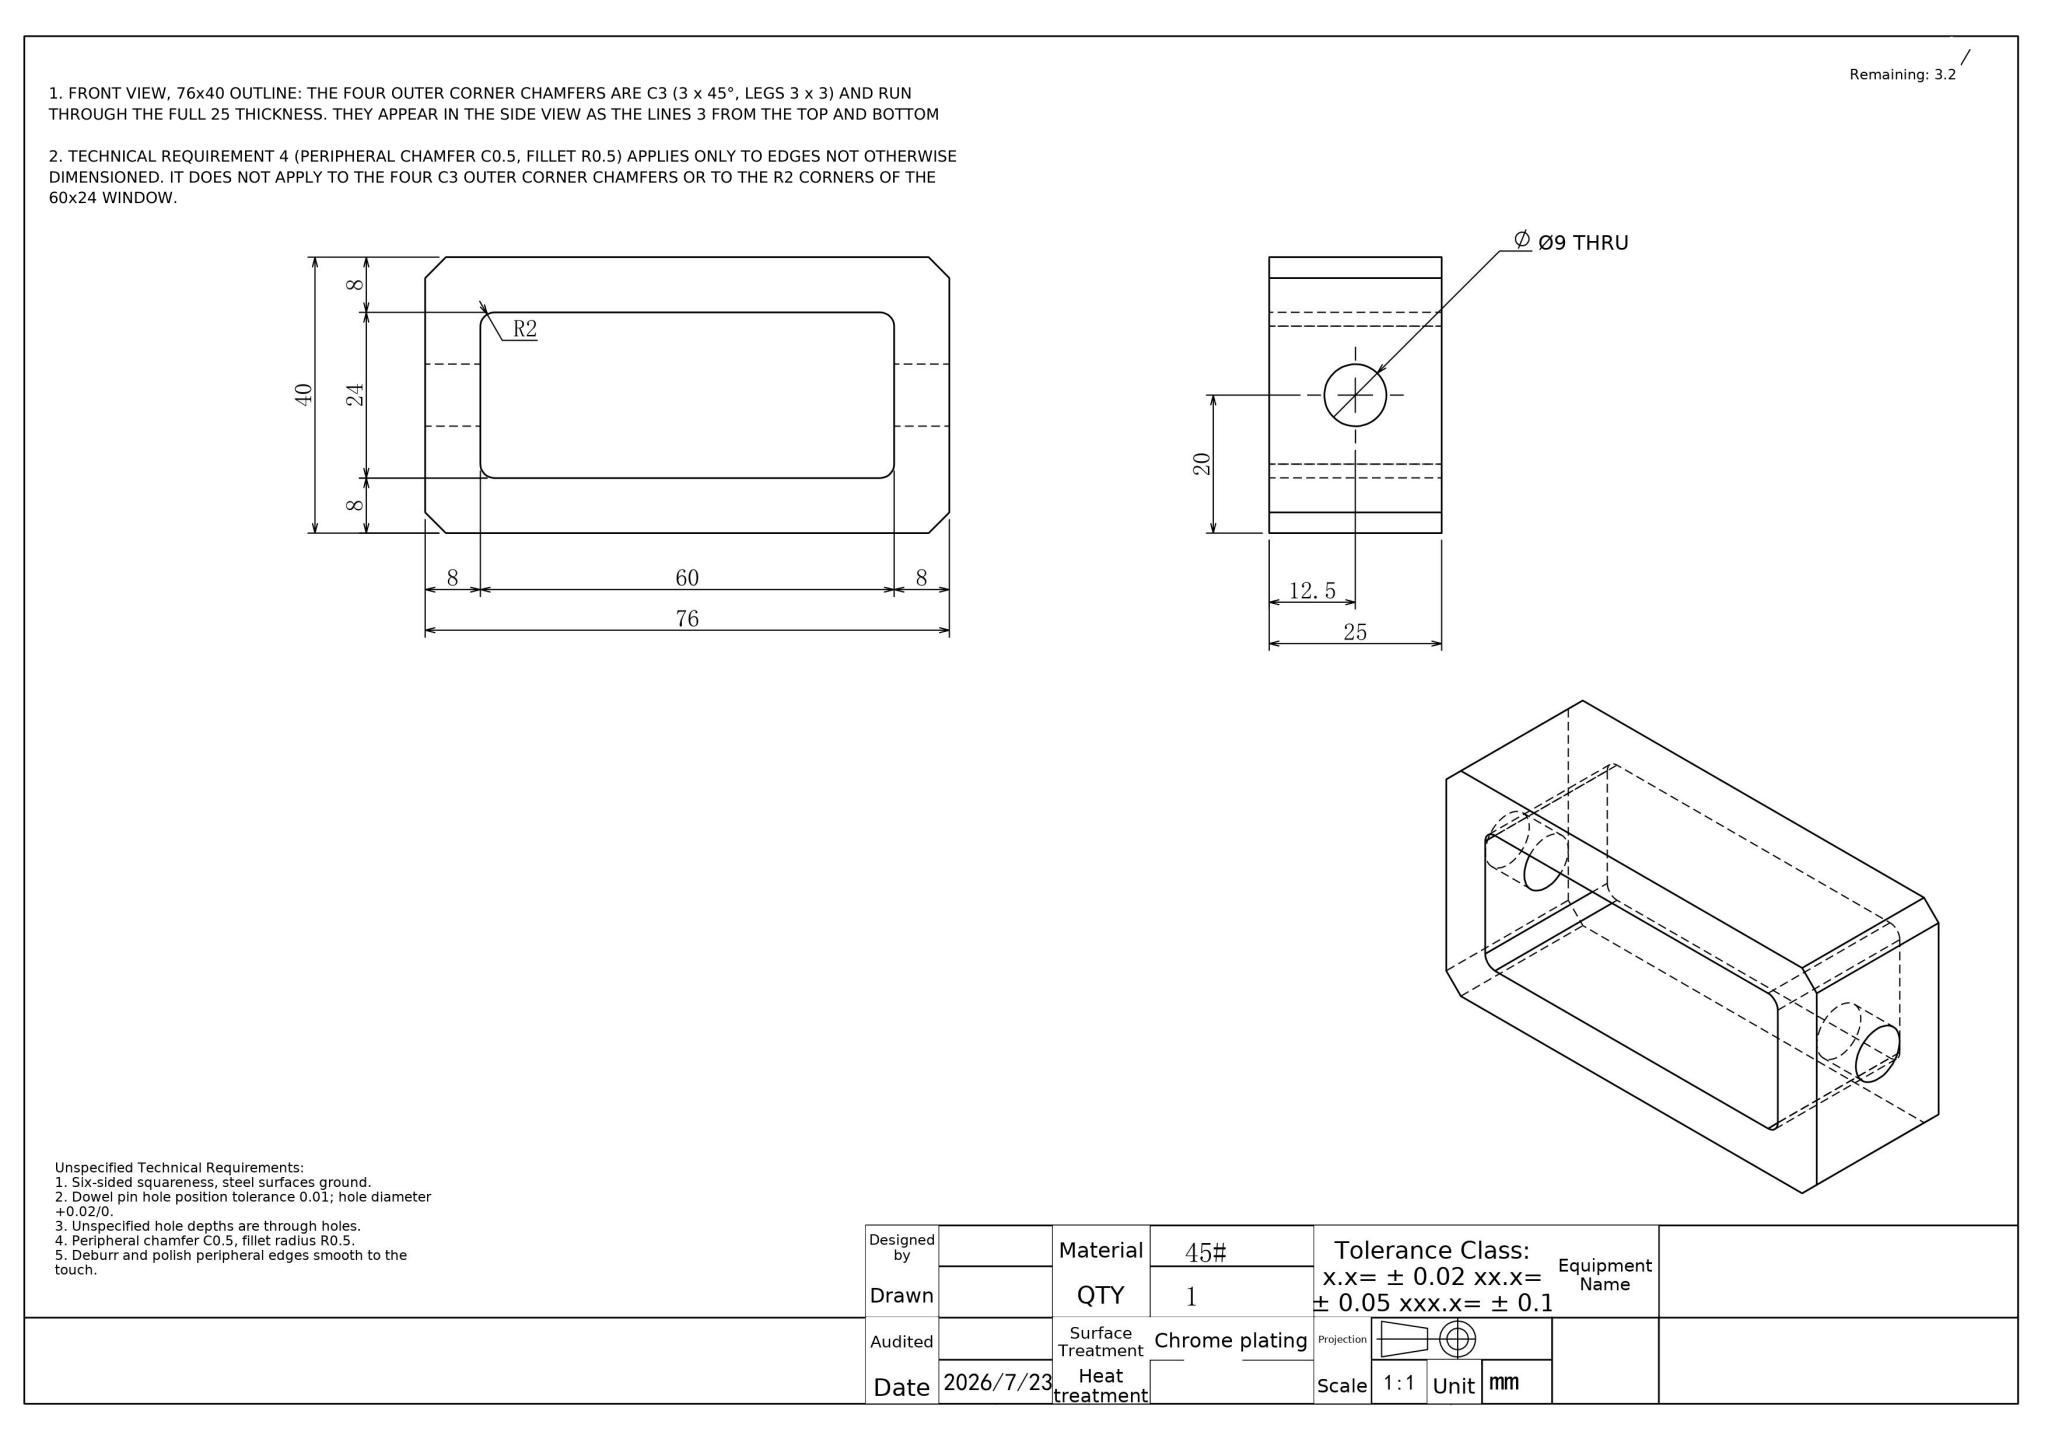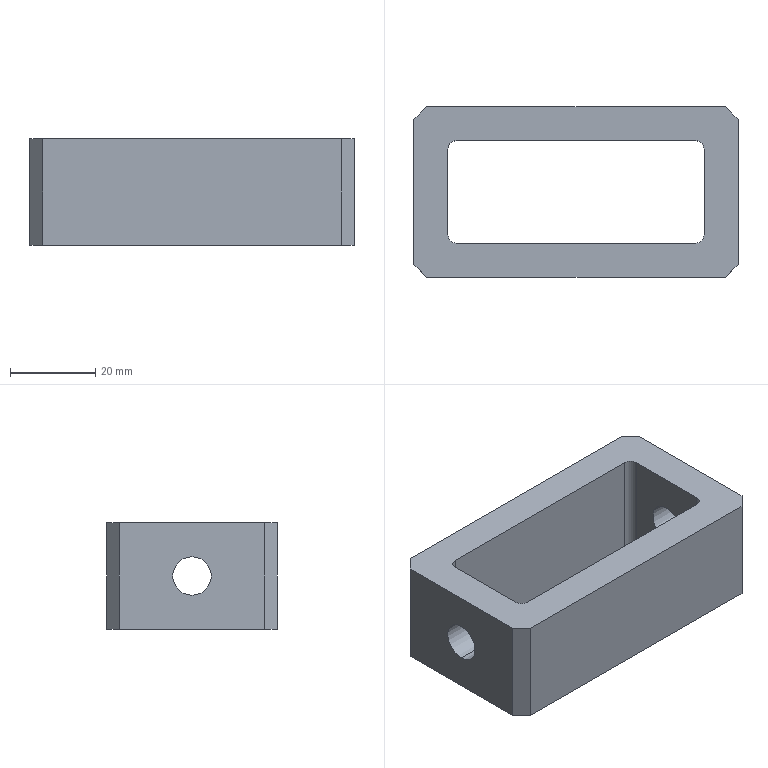Part | NX | mm | Rectangular Slotted Mounting Block | 1 solid | 22 faces | box 76 x 40 x 25 mm | volume 38618 mm3 | plane 14 | cylinder 8 | commonest cylinder face diameters 9 x4 4 x4
STEP:
#1=CARTESIAN_POINT('',(-38.,0.,17.));
#2=VERTEX_POINT('',#1);
#3=CARTESIAN_POINT('',(-38.,0.,8.));
#4=VERTEX_POINT('',#3);
#5=CARTESIAN_POINT('',(-38.,0.,12.5));
#6=DIRECTION('',(1.,0.,0.));
#7=DIRECTION('',(0.,0.,-1.));
#8=AXIS2_PLACEMENT_3D('',#5,#6,#7);
#9=CIRCLE('',#8,4.5);
#10=EDGE_CURVE('',#2,#4,#9,.T.);
#11=ORIENTED_EDGE('',*,*,#10,.F.);
#12=CARTESIAN_POINT('',(-30.,0.,17.));
#13=VERTEX_POINT('',#12);
#14=CARTESIAN_POINT('',(-38.,0.,17.));
#15=DIRECTION('',(1.,0.,0.));
#16=VECTOR('',#15,1000.);
#17=LINE('',#14,#16);
#18=EDGE_CURVE('',#2,#13,#17,.T.);
#19=ORIENTED_EDGE('',*,*,#18,.T.);
#20=CARTESIAN_POINT('',(-30.,0.,8.));
#21=VERTEX_POINT('',#20);
#22=CARTESIAN_POINT('',(-30.,0.,12.5));
#23=DIRECTION('',(1.,0.,0.));
#24=DIRECTION('',(0.,0.,-1.));
#25=AXIS2_PLACEMENT_3D('',#22,#23,#24);
#26=CIRCLE('',#25,4.5);
#27=EDGE_CURVE('',#13,#21,#26,.T.);
#28=ORIENTED_EDGE('',*,*,#27,.T.);
#29=CARTESIAN_POINT('',(-38.,0.,8.));
#30=DIRECTION('',(1.,0.,0.));
#31=VECTOR('',#30,1000.);
#32=LINE('',#29,#31);
#33=EDGE_CURVE('',#4,#21,#32,.T.);
#34=ORIENTED_EDGE('',*,*,#33,.F.);
#35=EDGE_LOOP('',(#11,#19,#28,#34));
#36=FACE_OUTER_BOUND('',#35,.T.);
#37=CARTESIAN_POINT('',(-38.,0.,12.5));
#38=DIRECTION('',(1.,0.,0.));
#39=DIRECTION('',(0.,0.,-1.));
#40=AXIS2_PLACEMENT_3D('',#37,#38,#39);
#41=CYLINDRICAL_SURFACE('',#40,4.5);
#42=ADVANCED_FACE('',(#36),#41,.F.);
#43=CARTESIAN_POINT('',(30.,0.,8.));
#44=VERTEX_POINT('',#43);
#45=CARTESIAN_POINT('',(30.,0.,17.));
#46=VERTEX_POINT('',#45);
#47=CARTESIAN_POINT('',(30.,0.,12.5));
#48=DIRECTION('',(-1.,0.,0.));
#49=DIRECTION('',(0.,0.,-1.));
#50=AXIS2_PLACEMENT_3D('',#47,#48,#49);
#51=CIRCLE('',#50,4.5);
#52=EDGE_CURVE('',#44,#46,#51,.T.);
#53=ORIENTED_EDGE('',*,*,#52,.T.);
#54=CARTESIAN_POINT('',(38.,0.,17.));
#55=VERTEX_POINT('',#54);
#56=CARTESIAN_POINT('',(-38.001,0.,17.));
#57=DIRECTION('',(1.,0.,0.));
#58=VECTOR('',#57,1000.);
#59=LINE('',#56,#58);
#60=EDGE_CURVE('',#46,#55,#59,.T.);
#61=ORIENTED_EDGE('',*,*,#60,.T.);
#62=CARTESIAN_POINT('',(38.,0.,8.));
#63=VERTEX_POINT('',#62);
#64=CARTESIAN_POINT('',(38.,0.,12.5));
#65=DIRECTION('',(1.,0.,0.));
#66=DIRECTION('',(0.,0.,-1.));
#67=AXIS2_PLACEMENT_3D('',#64,#65,#66);
#68=CIRCLE('',#67,4.5);
#69=EDGE_CURVE('',#55,#63,#68,.T.);
#70=ORIENTED_EDGE('',*,*,#69,.T.);
#71=CARTESIAN_POINT('',(-38.001,0.,8.));
#72=DIRECTION('',(1.,0.,0.));
#73=VECTOR('',#72,1000.);
#74=LINE('',#71,#73);
#75=EDGE_CURVE('',#44,#63,#74,.T.);
#76=ORIENTED_EDGE('',*,*,#75,.F.);
#77=EDGE_LOOP('',(#53,#61,#70,#76));
#78=FACE_OUTER_BOUND('',#77,.T.);
#79=CARTESIAN_POINT('',(-38.001,0.,12.5));
#80=DIRECTION('',(1.,0.,0.));
#81=DIRECTION('',(0.,0.,-1.));
#82=AXIS2_PLACEMENT_3D('',#79,#80,#81);
#83=CYLINDRICAL_SURFACE('',#82,4.5);
#84=ADVANCED_FACE('',(#78),#83,.F.);
#85=CARTESIAN_POINT('',(38.,0.,12.5));
#86=DIRECTION('',(1.,0.,0.));
#87=DIRECTION('',(0.,0.,-1.));
#88=AXIS2_PLACEMENT_3D('',#85,#86,#87);
#89=CIRCLE('',#88,4.5);
#90=EDGE_CURVE('',#63,#55,#89,.T.);
#91=ORIENTED_EDGE('',*,*,#90,.F.);
#92=ORIENTED_EDGE('',*,*,#69,.F.);
#93=EDGE_LOOP('',(#91,#92));
#94=FACE_BOUND('',#93,.T.);
#95=CARTESIAN_POINT('',(38.,-17.,25.));
#96=VERTEX_POINT('',#95);
#97=CARTESIAN_POINT('',(38.,17.,25.));
#98=VERTEX_POINT('',#97);
#99=CARTESIAN_POINT('',(38.,-20.,25.));
#100=DIRECTION('',(0.,1.,0.));
#101=VECTOR('',#100,1000.);
#102=LINE('',#99,#101);
#103=EDGE_CURVE('',#96,#98,#102,.T.);
#104=ORIENTED_EDGE('',*,*,#103,.F.);
#105=CARTESIAN_POINT('',(38.,-17.,0.));
#106=VERTEX_POINT('',#105);
#107=CARTESIAN_POINT('',(38.,-17.,25.));
#108=DIRECTION('',(0.,0.,-1.));
#109=VECTOR('',#108,1000.);
#110=LINE('',#107,#109);
#111=EDGE_CURVE('',#96,#106,#110,.T.);
#112=ORIENTED_EDGE('',*,*,#111,.T.);
#113=CARTESIAN_POINT('',(38.,17.,0.));
#114=VERTEX_POINT('',#113);
#115=CARTESIAN_POINT('',(38.,-20.,0.));
#116=DIRECTION('',(0.,1.,0.));
#117=VECTOR('',#116,1000.);
#118=LINE('',#115,#117);
#119=EDGE_CURVE('',#106,#114,#118,.T.);
#120=ORIENTED_EDGE('',*,*,#119,.T.);
#121=CARTESIAN_POINT('',(38.,17.,25.));
#122=DIRECTION('',(0.,0.,1.));
#123=VECTOR('',#122,1000.);
#124=LINE('',#121,#123);
#125=EDGE_CURVE('',#114,#98,#124,.T.);
#126=ORIENTED_EDGE('',*,*,#125,.T.);
#127=EDGE_LOOP('',(#104,#112,#120,#126));
#128=FACE_OUTER_BOUND('',#127,.T.);
#129=CARTESIAN_POINT('',(38.,-20.,25.));
#130=DIRECTION('',(-1.,0.,0.));
#131=DIRECTION('',(0.,0.,1.));
#132=AXIS2_PLACEMENT_3D('',#129,#130,#131);
#133=PLANE('',#132);
#134=ADVANCED_FACE('',(#94,#128),#133,.F.);
#135=CARTESIAN_POINT('',(35.,20.,0.));
#136=VERTEX_POINT('',#135);
#137=CARTESIAN_POINT('',(-35.,20.,0.));
#138=VERTEX_POINT('',#137);
#139=CARTESIAN_POINT('',(-38.,20.,0.));
#140=DIRECTION('',(-1.,0.,0.));
#141=VECTOR('',#140,1000.);
#142=LINE('',#139,#141);
#143=EDGE_CURVE('',#136,#138,#142,.T.);
#144=ORIENTED_EDGE('',*,*,#143,.T.);
#145=CARTESIAN_POINT('',(-35.,20.,25.));
#146=VERTEX_POINT('',#145);
#147=CARTESIAN_POINT('',(-35.,20.,25.));
#148=DIRECTION('',(0.,0.,1.));
#149=VECTOR('',#148,1000.);
#150=LINE('',#147,#149);
#151=EDGE_CURVE('',#138,#146,#150,.T.);
#152=ORIENTED_EDGE('',*,*,#151,.T.);
#153=CARTESIAN_POINT('',(35.,20.,25.));
#154=VERTEX_POINT('',#153);
#155=CARTESIAN_POINT('',(-38.,20.,25.));
#156=DIRECTION('',(-1.,0.,0.));
#157=VECTOR('',#156,1000.);
#158=LINE('',#155,#157);
#159=EDGE_CURVE('',#154,#146,#158,.T.);
#160=ORIENTED_EDGE('',*,*,#159,.F.);
#161=CARTESIAN_POINT('',(35.,20.,25.));
#162=DIRECTION('',(0.,0.,-1.));
#163=VECTOR('',#162,1000.);
#164=LINE('',#161,#163);
#165=EDGE_CURVE('',#154,#136,#164,.T.);
#166=ORIENTED_EDGE('',*,*,#165,.T.);
#167=EDGE_LOOP('',(#144,#152,#160,#166));
#168=FACE_OUTER_BOUND('',#167,.T.);
#169=CARTESIAN_POINT('',(-38.,20.,25.));
#170=DIRECTION('',(0.,-1.,0.));
#171=DIRECTION('',(0.,0.,-1.));
#172=AXIS2_PLACEMENT_3D('',#169,#170,#171);
#173=PLANE('',#172);
#174=ADVANCED_FACE('',(#168),#173,.F.);
#175=CARTESIAN_POINT('',(-38.,0.,12.5));
#176=DIRECTION('',(1.,0.,0.));
#177=DIRECTION('',(0.,0.,-1.));
#178=AXIS2_PLACEMENT_3D('',#175,#176,#177);
#179=CIRCLE('',#178,4.5);
#180=EDGE_CURVE('',#4,#2,#179,.T.);
#181=ORIENTED_EDGE('',*,*,#180,.T.);
#182=ORIENTED_EDGE('',*,*,#10,.T.);
#183=EDGE_LOOP('',(#181,#182));
#184=FACE_BOUND('',#183,.T.);
#185=CARTESIAN_POINT('',(-38.,17.,0.));
#186=VERTEX_POINT('',#185);
#187=CARTESIAN_POINT('',(-38.,-17.,0.));
#188=VERTEX_POINT('',#187);
#189=CARTESIAN_POINT('',(-38.,-20.,0.));
#190=DIRECTION('',(0.,-1.,0.));
#191=VECTOR('',#190,1000.);
#192=LINE('',#189,#191);
#193=EDGE_CURVE('',#186,#188,#192,.T.);
#194=ORIENTED_EDGE('',*,*,#193,.T.);
#195=CARTESIAN_POINT('',(-38.,-17.,25.));
#196=VERTEX_POINT('',#195);
#197=CARTESIAN_POINT('',(-38.,-17.,25.));
#198=DIRECTION('',(0.,0.,1.));
#199=VECTOR('',#198,1000.);
#200=LINE('',#197,#199);
#201=EDGE_CURVE('',#188,#196,#200,.T.);
#202=ORIENTED_EDGE('',*,*,#201,.T.);
#203=CARTESIAN_POINT('',(-38.,17.,25.));
#204=VERTEX_POINT('',#203);
#205=CARTESIAN_POINT('',(-38.,-20.,25.));
#206=DIRECTION('',(0.,-1.,0.));
#207=VECTOR('',#206,1000.);
#208=LINE('',#205,#207);
#209=EDGE_CURVE('',#204,#196,#208,.T.);
#210=ORIENTED_EDGE('',*,*,#209,.F.);
#211=CARTESIAN_POINT('',(-38.,17.,25.));
#212=DIRECTION('',(0.,0.,-1.));
#213=VECTOR('',#212,1000.);
#214=LINE('',#211,#213);
#215=EDGE_CURVE('',#204,#186,#214,.T.);
#216=ORIENTED_EDGE('',*,*,#215,.T.);
#217=EDGE_LOOP('',(#194,#202,#210,#216));
#218=FACE_OUTER_BOUND('',#217,.T.);
#219=CARTESIAN_POINT('',(-38.,-20.,25.));
#220=DIRECTION('',(1.,0.,0.));
#221=DIRECTION('',(0.,0.,-1.));
#222=AXIS2_PLACEMENT_3D('',#219,#220,#221);
#223=PLANE('',#222);
#224=ADVANCED_FACE('',(#184,#218),#223,.F.);
#225=CARTESIAN_POINT('',(-35.,-20.,25.));
#226=VERTEX_POINT('',#225);
#227=CARTESIAN_POINT('',(35.,-20.,25.));
#228=VERTEX_POINT('',#227);
#229=CARTESIAN_POINT('',(-38.,-20.,25.));
#230=DIRECTION('',(1.,0.,0.));
#231=VECTOR('',#230,1000.);
#232=LINE('',#229,#231);
#233=EDGE_CURVE('',#226,#228,#232,.T.);
#234=ORIENTED_EDGE('',*,*,#233,.F.);
#235=CARTESIAN_POINT('',(-35.,-20.,0.));
#236=VERTEX_POINT('',#235);
#237=CARTESIAN_POINT('',(-35.,-20.,25.));
#238=DIRECTION('',(0.,0.,-1.));
#239=VECTOR('',#238,1000.);
#240=LINE('',#237,#239);
#241=EDGE_CURVE('',#226,#236,#240,.T.);
#242=ORIENTED_EDGE('',*,*,#241,.T.);
#243=CARTESIAN_POINT('',(35.,-20.,0.));
#244=VERTEX_POINT('',#243);
#245=CARTESIAN_POINT('',(-38.,-20.,0.));
#246=DIRECTION('',(1.,0.,0.));
#247=VECTOR('',#246,1000.);
#248=LINE('',#245,#247);
#249=EDGE_CURVE('',#236,#244,#248,.T.);
#250=ORIENTED_EDGE('',*,*,#249,.T.);
#251=CARTESIAN_POINT('',(35.,-20.,25.));
#252=DIRECTION('',(0.,0.,1.));
#253=VECTOR('',#252,1000.);
#254=LINE('',#251,#253);
#255=EDGE_CURVE('',#244,#228,#254,.T.);
#256=ORIENTED_EDGE('',*,*,#255,.T.);
#257=EDGE_LOOP('',(#234,#242,#250,#256));
#258=FACE_OUTER_BOUND('',#257,.T.);
#259=CARTESIAN_POINT('',(-38.,-20.,25.));
#260=DIRECTION('',(0.,1.,0.));
#261=DIRECTION('',(0.,0.,1.));
#262=AXIS2_PLACEMENT_3D('',#259,#260,#261);
#263=PLANE('',#262);
#264=ADVANCED_FACE('',(#258),#263,.F.);
#265=CARTESIAN_POINT('',(28.,12.,25.));
#266=VERTEX_POINT('',#265);
#267=CARTESIAN_POINT('',(-28.,12.,25.));
#268=VERTEX_POINT('',#267);
#269=CARTESIAN_POINT('',(-30.,12.,25.));
#270=DIRECTION('',(-1.,0.,0.));
#271=VECTOR('',#270,1000.);
#272=LINE('',#269,#271);
#273=EDGE_CURVE('',#266,#268,#272,.T.);
#274=ORIENTED_EDGE('',*,*,#273,.F.);
#275=CARTESIAN_POINT('',(30.,10.,25.));
#276=VERTEX_POINT('',#275);
#277=CARTESIAN_POINT('',(28.,10.,25.));
#278=DIRECTION('',(0.,0.,-1.));
#279=DIRECTION('',(-1.,0.,0.));
#280=AXIS2_PLACEMENT_3D('',#277,#278,#279);
#281=CIRCLE('',#280,2.);
#282=EDGE_CURVE('',#266,#276,#281,.T.);
#283=ORIENTED_EDGE('',*,*,#282,.T.);
#284=CARTESIAN_POINT('',(30.,-10.,25.));
#285=VERTEX_POINT('',#284);
#286=CARTESIAN_POINT('',(30.,-12.,25.));
#287=DIRECTION('',(0.,1.,0.));
#288=VECTOR('',#287,1000.);
#289=LINE('',#286,#288);
#290=EDGE_CURVE('',#285,#276,#289,.T.);
#291=ORIENTED_EDGE('',*,*,#290,.F.);
#292=CARTESIAN_POINT('',(28.,-12.,25.));
#293=VERTEX_POINT('',#292);
#294=CARTESIAN_POINT('',(28.,-10.,25.));
#295=DIRECTION('',(0.,0.,-1.));
#296=DIRECTION('',(-1.,0.,0.));
#297=AXIS2_PLACEMENT_3D('',#294,#295,#296);
#298=CIRCLE('',#297,2.);
#299=EDGE_CURVE('',#285,#293,#298,.T.);
#300=ORIENTED_EDGE('',*,*,#299,.T.);
#301=CARTESIAN_POINT('',(-28.,-12.,25.));
#302=VERTEX_POINT('',#301);
#303=CARTESIAN_POINT('',(-30.,-12.,25.));
#304=DIRECTION('',(1.,0.,0.));
#305=VECTOR('',#304,1000.);
#306=LINE('',#303,#305);
#307=EDGE_CURVE('',#302,#293,#306,.T.);
#308=ORIENTED_EDGE('',*,*,#307,.F.);
#309=CARTESIAN_POINT('',(-30.,-10.,25.));
#310=VERTEX_POINT('',#309);
#311=CARTESIAN_POINT('',(-28.,-10.,25.));
#312=DIRECTION('',(0.,0.,-1.));
#313=DIRECTION('',(-1.,0.,0.));
#314=AXIS2_PLACEMENT_3D('',#311,#312,#313);
#315=CIRCLE('',#314,2.);
#316=EDGE_CURVE('',#302,#310,#315,.T.);
#317=ORIENTED_EDGE('',*,*,#316,.T.);
#318=CARTESIAN_POINT('',(-30.,10.,25.));
#319=VERTEX_POINT('',#318);
#320=CARTESIAN_POINT('',(-30.,-12.,25.));
#321=DIRECTION('',(0.,-1.,0.));
#322=VECTOR('',#321,1000.);
#323=LINE('',#320,#322);
#324=EDGE_CURVE('',#319,#310,#323,.T.);
#325=ORIENTED_EDGE('',*,*,#324,.F.);
#326=CARTESIAN_POINT('',(-28.,10.,25.));
#327=DIRECTION('',(0.,0.,-1.));
#328=DIRECTION('',(-1.,0.,0.));
#329=AXIS2_PLACEMENT_3D('',#326,#327,#328);
#330=CIRCLE('',#329,2.);
#331=EDGE_CURVE('',#319,#268,#330,.T.);
#332=ORIENTED_EDGE('',*,*,#331,.T.);
#333=EDGE_LOOP('',(#274,#283,#291,#300,#308,#317,#325,#332));
#334=FACE_BOUND('',#333,.T.);
#335=ORIENTED_EDGE('',*,*,#209,.T.);
#336=CARTESIAN_POINT('',(-35.,-20.,25.));
#337=DIRECTION('',(0.7071,-0.7071,0.));
#338=VECTOR('',#337,1000.);
#339=LINE('',#336,#338);
#340=EDGE_CURVE('',#196,#226,#339,.T.);
#341=ORIENTED_EDGE('',*,*,#340,.T.);
#342=ORIENTED_EDGE('',*,*,#233,.T.);
#343=CARTESIAN_POINT('',(38.,-17.,25.));
#344=DIRECTION('',(0.7071,0.7071,0.));
#345=VECTOR('',#344,1000.);
#346=LINE('',#343,#345);
#347=EDGE_CURVE('',#228,#96,#346,.T.);
#348=ORIENTED_EDGE('',*,*,#347,.T.);
#349=ORIENTED_EDGE('',*,*,#103,.T.);
#350=CARTESIAN_POINT('',(35.,20.,25.));
#351=DIRECTION('',(-0.7071,0.7071,0.));
#352=VECTOR('',#351,1000.);
#353=LINE('',#350,#352);
#354=EDGE_CURVE('',#98,#154,#353,.T.);
#355=ORIENTED_EDGE('',*,*,#354,.T.);
#356=ORIENTED_EDGE('',*,*,#159,.T.);
#357=CARTESIAN_POINT('',(-38.,17.,25.));
#358=DIRECTION('',(-0.7071,-0.7071,0.));
#359=VECTOR('',#358,1000.);
#360=LINE('',#357,#359);
#361=EDGE_CURVE('',#146,#204,#360,.T.);
#362=ORIENTED_EDGE('',*,*,#361,.T.);
#363=EDGE_LOOP('',(#335,#341,#342,#348,#349,#355,#356,#362));
#364=FACE_OUTER_BOUND('',#363,.T.);
#365=CARTESIAN_POINT('',(0.,0.,25.));
#366=DIRECTION('',(0.,0.,-1.));
#367=DIRECTION('',(-1.,0.,0.));
#368=AXIS2_PLACEMENT_3D('',#365,#366,#367);
#369=PLANE('',#368);
#370=ADVANCED_FACE('',(#334,#364),#369,.F.);
#371=CARTESIAN_POINT('',(-28.,-12.,0.));
#372=VERTEX_POINT('',#371);
#373=CARTESIAN_POINT('',(28.,-12.,0.));
#374=VERTEX_POINT('',#373);
#375=CARTESIAN_POINT('',(-30.,-12.,0.));
#376=DIRECTION('',(1.,0.,0.));
#377=VECTOR('',#376,1000.);
#378=LINE('',#375,#377);
#379=EDGE_CURVE('',#372,#374,#378,.T.);
#380=ORIENTED_EDGE('',*,*,#379,.T.);
#381=CARTESIAN_POINT('',(30.,-10.,0.));
#382=VERTEX_POINT('',#381);
#383=CARTESIAN_POINT('',(28.,-10.,0.));
#384=DIRECTION('',(0.,0.,1.));
#385=DIRECTION('',(-1.,0.,0.));
#386=AXIS2_PLACEMENT_3D('',#383,#384,#385);
#387=CIRCLE('',#386,2.);
#388=EDGE_CURVE('',#374,#382,#387,.T.);
#389=ORIENTED_EDGE('',*,*,#388,.T.);
#390=CARTESIAN_POINT('',(30.,10.,0.));
#391=VERTEX_POINT('',#390);
#392=CARTESIAN_POINT('',(30.,-12.,0.));
#393=DIRECTION('',(0.,1.,0.));
#394=VECTOR('',#393,1000.);
#395=LINE('',#392,#394);
#396=EDGE_CURVE('',#382,#391,#395,.T.);
#397=ORIENTED_EDGE('',*,*,#396,.T.);
#398=CARTESIAN_POINT('',(28.,12.,0.));
#399=VERTEX_POINT('',#398);
#400=CARTESIAN_POINT('',(28.,10.,0.));
#401=DIRECTION('',(0.,0.,1.));
#402=DIRECTION('',(-1.,0.,0.));
#403=AXIS2_PLACEMENT_3D('',#400,#401,#402);
#404=CIRCLE('',#403,2.);
#405=EDGE_CURVE('',#391,#399,#404,.T.);
#406=ORIENTED_EDGE('',*,*,#405,.T.);
#407=CARTESIAN_POINT('',(-28.,12.,0.));
#408=VERTEX_POINT('',#407);
#409=CARTESIAN_POINT('',(-30.,12.,0.));
#410=DIRECTION('',(-1.,0.,0.));
#411=VECTOR('',#410,1000.);
#412=LINE('',#409,#411);
#413=EDGE_CURVE('',#399,#408,#412,.T.);
#414=ORIENTED_EDGE('',*,*,#413,.T.);
#415=CARTESIAN_POINT('',(-30.,10.,0.));
#416=VERTEX_POINT('',#415);
#417=CARTESIAN_POINT('',(-28.,10.,0.));
#418=DIRECTION('',(0.,0.,1.));
#419=DIRECTION('',(-1.,0.,0.));
#420=AXIS2_PLACEMENT_3D('',#417,#418,#419);
#421=CIRCLE('',#420,2.);
#422=EDGE_CURVE('',#408,#416,#421,.T.);
#423=ORIENTED_EDGE('',*,*,#422,.T.);
#424=CARTESIAN_POINT('',(-30.,-10.,0.));
#425=VERTEX_POINT('',#424);
#426=CARTESIAN_POINT('',(-30.,-12.,0.));
#427=DIRECTION('',(0.,-1.,0.));
#428=VECTOR('',#427,1000.);
#429=LINE('',#426,#428);
#430=EDGE_CURVE('',#416,#425,#429,.T.);
#431=ORIENTED_EDGE('',*,*,#430,.T.);
#432=CARTESIAN_POINT('',(-28.,-10.,0.));
#433=DIRECTION('',(0.,0.,1.));
#434=DIRECTION('',(-1.,0.,0.));
#435=AXIS2_PLACEMENT_3D('',#432,#433,#434);
#436=CIRCLE('',#435,2.);
#437=EDGE_CURVE('',#425,#372,#436,.T.);
#438=ORIENTED_EDGE('',*,*,#437,.T.);
#439=EDGE_LOOP('',(#380,#389,#397,#406,#414,#423,#431,#438));
#440=FACE_BOUND('',#439,.T.);
#441=ORIENTED_EDGE('',*,*,#249,.F.);
#442=CARTESIAN_POINT('',(-27.5,-27.5,0.));
#443=DIRECTION('',(-0.7071,0.7071,0.));
#444=VECTOR('',#443,1000.);
#445=LINE('',#442,#444);
#446=EDGE_CURVE('',#236,#188,#445,.T.);
#447=ORIENTED_EDGE('',*,*,#446,.T.);
#448=ORIENTED_EDGE('',*,*,#193,.F.);
#449=CARTESIAN_POINT('',(-27.5,27.5,0.));
#450=DIRECTION('',(0.7071,0.7071,0.));
#451=VECTOR('',#450,1000.);
#452=LINE('',#449,#451);
#453=EDGE_CURVE('',#186,#138,#452,.T.);
#454=ORIENTED_EDGE('',*,*,#453,.T.);
#455=ORIENTED_EDGE('',*,*,#143,.F.);
#456=CARTESIAN_POINT('',(27.5,27.5,0.));
#457=DIRECTION('',(0.7071,-0.7071,0.));
#458=VECTOR('',#457,1000.);
#459=LINE('',#456,#458);
#460=EDGE_CURVE('',#136,#114,#459,.T.);
#461=ORIENTED_EDGE('',*,*,#460,.T.);
#462=ORIENTED_EDGE('',*,*,#119,.F.);
#463=CARTESIAN_POINT('',(27.5,-27.5,0.));
#464=DIRECTION('',(-0.7071,-0.7071,0.));
#465=VECTOR('',#464,1000.);
#466=LINE('',#463,#465);
#467=EDGE_CURVE('',#106,#244,#466,.T.);
#468=ORIENTED_EDGE('',*,*,#467,.T.);
#469=EDGE_LOOP('',(#441,#447,#448,#454,#455,#461,#462,#468));
#470=FACE_OUTER_BOUND('',#469,.T.);
#471=CARTESIAN_POINT('',(0.,0.,0.));
#472=DIRECTION('',(0.,0.,-1.));
#473=DIRECTION('',(-1.,0.,0.));
#474=AXIS2_PLACEMENT_3D('',#471,#472,#473);
#475=PLANE('',#474);
#476=ADVANCED_FACE('',(#440,#470),#475,.T.);
#477=ORIENTED_EDGE('',*,*,#52,.F.);
#478=CARTESIAN_POINT('',(30.,0.,12.5));
#479=DIRECTION('',(-1.,0.,0.));
#480=DIRECTION('',(0.,0.,-1.));
#481=AXIS2_PLACEMENT_3D('',#478,#479,#480);
#482=CIRCLE('',#481,4.5);
#483=EDGE_CURVE('',#46,#44,#482,.T.);
#484=ORIENTED_EDGE('',*,*,#483,.F.);
#485=EDGE_LOOP('',(#477,#484));
#486=FACE_BOUND('',#485,.T.);
#487=ORIENTED_EDGE('',*,*,#290,.T.);
#488=CARTESIAN_POINT('',(30.,10.,0.));
#489=DIRECTION('',(0.,0.,-1.));
#490=VECTOR('',#489,1000.);
#491=LINE('',#488,#490);
#492=EDGE_CURVE('',#276,#391,#491,.T.);
#493=ORIENTED_EDGE('',*,*,#492,.T.);
#494=ORIENTED_EDGE('',*,*,#396,.F.);
#495=CARTESIAN_POINT('',(30.,-10.,25.));
#496=DIRECTION('',(0.,0.,1.));
#497=VECTOR('',#496,1000.);
#498=LINE('',#495,#497);
#499=EDGE_CURVE('',#382,#285,#498,.T.);
#500=ORIENTED_EDGE('',*,*,#499,.T.);
#501=EDGE_LOOP('',(#487,#493,#494,#500));
#502=FACE_OUTER_BOUND('',#501,.T.);
#503=CARTESIAN_POINT('',(30.,-12.,0.));
#504=DIRECTION('',(1.,0.,0.));
#505=DIRECTION('',(0.,0.,-1.));
#506=AXIS2_PLACEMENT_3D('',#503,#504,#505);
#507=PLANE('',#506);
#508=ADVANCED_FACE('',(#486,#502),#507,.F.);
#509=ORIENTED_EDGE('',*,*,#307,.T.);
#510=CARTESIAN_POINT('',(28.,-12.,0.));
#511=DIRECTION('',(0.,0.,-1.));
#512=VECTOR('',#511,1000.);
#513=LINE('',#510,#512);
#514=EDGE_CURVE('',#293,#374,#513,.T.);
#515=ORIENTED_EDGE('',*,*,#514,.T.);
#516=ORIENTED_EDGE('',*,*,#379,.F.);
#517=CARTESIAN_POINT('',(-28.,-12.,25.));
#518=DIRECTION('',(0.,0.,1.));
#519=VECTOR('',#518,1000.);
#520=LINE('',#517,#519);
#521=EDGE_CURVE('',#372,#302,#520,.T.);
#522=ORIENTED_EDGE('',*,*,#521,.T.);
#523=EDGE_LOOP('',(#509,#515,#516,#522));
#524=FACE_OUTER_BOUND('',#523,.T.);
#525=CARTESIAN_POINT('',(-30.,-12.,0.));
#526=DIRECTION('',(0.,-1.,0.));
#527=DIRECTION('',(0.,0.,-1.));
#528=AXIS2_PLACEMENT_3D('',#525,#526,#527);
#529=PLANE('',#528);
#530=ADVANCED_FACE('',(#524),#529,.F.);
#531=CARTESIAN_POINT('',(-30.,0.,12.5));
#532=DIRECTION('',(1.,0.,0.));
#533=DIRECTION('',(0.,0.,-1.));
#534=AXIS2_PLACEMENT_3D('',#531,#532,#533);
#535=CIRCLE('',#534,4.5);
#536=EDGE_CURVE('',#21,#13,#535,.T.);
#537=ORIENTED_EDGE('',*,*,#536,.F.);
#538=ORIENTED_EDGE('',*,*,#27,.F.);
#539=EDGE_LOOP('',(#537,#538));
#540=FACE_BOUND('',#539,.T.);
#541=ORIENTED_EDGE('',*,*,#324,.T.);
#542=CARTESIAN_POINT('',(-30.,-10.,0.));
#543=DIRECTION('',(0.,0.,-1.));
#544=VECTOR('',#543,1000.);
#545=LINE('',#542,#544);
#546=EDGE_CURVE('',#310,#425,#545,.T.);
#547=ORIENTED_EDGE('',*,*,#546,.T.);
#548=ORIENTED_EDGE('',*,*,#430,.F.);
#549=CARTESIAN_POINT('',(-30.,10.,25.));
#550=DIRECTION('',(0.,0.,1.));
#551=VECTOR('',#550,1000.);
#552=LINE('',#549,#551);
#553=EDGE_CURVE('',#416,#319,#552,.T.);
#554=ORIENTED_EDGE('',*,*,#553,.T.);
#555=EDGE_LOOP('',(#541,#547,#548,#554));
#556=FACE_OUTER_BOUND('',#555,.T.);
#557=CARTESIAN_POINT('',(-30.,-12.,0.));
#558=DIRECTION('',(-1.,0.,0.));
#559=DIRECTION('',(0.,0.,1.));
#560=AXIS2_PLACEMENT_3D('',#557,#558,#559);
#561=PLANE('',#560);
#562=ADVANCED_FACE('',(#540,#556),#561,.F.);
#563=ORIENTED_EDGE('',*,*,#413,.F.);
#564=CARTESIAN_POINT('',(28.,12.,25.));
#565=DIRECTION('',(0.,0.,1.));
#566=VECTOR('',#565,1000.);
#567=LINE('',#564,#566);
#568=EDGE_CURVE('',#399,#266,#567,.T.);
#569=ORIENTED_EDGE('',*,*,#568,.T.);
#570=ORIENTED_EDGE('',*,*,#273,.T.);
#571=CARTESIAN_POINT('',(-28.,12.,0.));
#572=DIRECTION('',(0.,0.,-1.));
#573=VECTOR('',#572,1000.);
#574=LINE('',#571,#573);
#575=EDGE_CURVE('',#268,#408,#574,.T.);
#576=ORIENTED_EDGE('',*,*,#575,.T.);
#577=EDGE_LOOP('',(#563,#569,#570,#576));
#578=FACE_OUTER_BOUND('',#577,.T.);
#579=CARTESIAN_POINT('',(-30.,12.,0.));
#580=DIRECTION('',(0.,1.,0.));
#581=DIRECTION('',(0.,0.,1.));
#582=AXIS2_PLACEMENT_3D('',#579,#580,#581);
#583=PLANE('',#582);
#584=ADVANCED_FACE('',(#578),#583,.F.);
#585=ORIENTED_EDGE('',*,*,#60,.F.);
#586=ORIENTED_EDGE('',*,*,#483,.T.);
#587=ORIENTED_EDGE('',*,*,#75,.T.);
#588=ORIENTED_EDGE('',*,*,#90,.T.);
#589=EDGE_LOOP('',(#585,#586,#587,#588));
#590=FACE_OUTER_BOUND('',#589,.T.);
#591=CARTESIAN_POINT('',(-38.001,0.,12.5));
#592=DIRECTION('',(1.,0.,0.));
#593=DIRECTION('',(0.,0.,-1.));
#594=AXIS2_PLACEMENT_3D('',#591,#592,#593);
#595=CYLINDRICAL_SURFACE('',#594,4.5);
#596=ADVANCED_FACE('',(#590),#595,.F.);
#597=ORIENTED_EDGE('',*,*,#18,.F.);
#598=ORIENTED_EDGE('',*,*,#180,.F.);
#599=ORIENTED_EDGE('',*,*,#33,.T.);
#600=ORIENTED_EDGE('',*,*,#536,.T.);
#601=EDGE_LOOP('',(#597,#598,#599,#600));
#602=FACE_OUTER_BOUND('',#601,.T.);
#603=CARTESIAN_POINT('',(-38.,0.,12.5));
#604=DIRECTION('',(1.,0.,0.));
#605=DIRECTION('',(0.,0.,-1.));
#606=AXIS2_PLACEMENT_3D('',#603,#604,#605);
#607=CYLINDRICAL_SURFACE('',#606,4.5);
#608=ADVANCED_FACE('',(#602),#607,.F.);
#609=ORIENTED_EDGE('',*,*,#405,.F.);
#610=ORIENTED_EDGE('',*,*,#492,.F.);
#611=ORIENTED_EDGE('',*,*,#282,.F.);
#612=ORIENTED_EDGE('',*,*,#568,.F.);
#613=EDGE_LOOP('',(#609,#610,#611,#612));
#614=FACE_OUTER_BOUND('',#613,.T.);
#615=CARTESIAN_POINT('',(28.,10.,0.));
#616=DIRECTION('',(0.,0.,-1.));
#617=DIRECTION('',(-1.,0.,0.));
#618=AXIS2_PLACEMENT_3D('',#615,#616,#617);
#619=CYLINDRICAL_SURFACE('',#618,2.);
#620=ADVANCED_FACE('',(#614),#619,.F.);
#621=ORIENTED_EDGE('',*,*,#388,.F.);
#622=ORIENTED_EDGE('',*,*,#514,.F.);
#623=ORIENTED_EDGE('',*,*,#299,.F.);
#624=ORIENTED_EDGE('',*,*,#499,.F.);
#625=EDGE_LOOP('',(#621,#622,#623,#624));
#626=FACE_OUTER_BOUND('',#625,.T.);
#627=CARTESIAN_POINT('',(28.,-10.,0.));
#628=DIRECTION('',(0.,0.,-1.));
#629=DIRECTION('',(-1.,0.,0.));
#630=AXIS2_PLACEMENT_3D('',#627,#628,#629);
#631=CYLINDRICAL_SURFACE('',#630,2.);
#632=ADVANCED_FACE('',(#626),#631,.F.);
#633=ORIENTED_EDGE('',*,*,#437,.F.);
#634=ORIENTED_EDGE('',*,*,#546,.F.);
#635=ORIENTED_EDGE('',*,*,#316,.F.);
#636=ORIENTED_EDGE('',*,*,#521,.F.);
#637=EDGE_LOOP('',(#633,#634,#635,#636));
#638=FACE_OUTER_BOUND('',#637,.T.);
#639=CARTESIAN_POINT('',(-28.,-10.,0.));
#640=DIRECTION('',(0.,0.,-1.));
#641=DIRECTION('',(-1.,0.,0.));
#642=AXIS2_PLACEMENT_3D('',#639,#640,#641);
#643=CYLINDRICAL_SURFACE('',#642,2.);
#644=ADVANCED_FACE('',(#638),#643,.F.);
#645=ORIENTED_EDGE('',*,*,#422,.F.);
#646=ORIENTED_EDGE('',*,*,#575,.F.);
#647=ORIENTED_EDGE('',*,*,#331,.F.);
#648=ORIENTED_EDGE('',*,*,#553,.F.);
#649=EDGE_LOOP('',(#645,#646,#647,#648));
#650=FACE_OUTER_BOUND('',#649,.T.);
#651=CARTESIAN_POINT('',(-28.,10.,0.));
#652=DIRECTION('',(0.,0.,-1.));
#653=DIRECTION('',(-1.,0.,0.));
#654=AXIS2_PLACEMENT_3D('',#651,#652,#653);
#655=CYLINDRICAL_SURFACE('',#654,2.);
#656=ADVANCED_FACE('',(#650),#655,.F.);
#657=ORIENTED_EDGE('',*,*,#340,.F.);
#658=ORIENTED_EDGE('',*,*,#201,.F.);
#659=ORIENTED_EDGE('',*,*,#446,.F.);
#660=ORIENTED_EDGE('',*,*,#241,.F.);
#661=EDGE_LOOP('',(#657,#658,#659,#660));
#662=FACE_OUTER_BOUND('',#661,.T.);
#663=CARTESIAN_POINT('',(-35.,-20.,25.));
#664=DIRECTION('',(0.7071,0.7071,0.));
#665=DIRECTION('',(0.,0.,-1.));
#666=AXIS2_PLACEMENT_3D('',#663,#664,#665);
#667=PLANE('',#666);
#668=ADVANCED_FACE('',(#662),#667,.F.);
#669=ORIENTED_EDGE('',*,*,#347,.F.);
#670=ORIENTED_EDGE('',*,*,#255,.F.);
#671=ORIENTED_EDGE('',*,*,#467,.F.);
#672=ORIENTED_EDGE('',*,*,#111,.F.);
#673=EDGE_LOOP('',(#669,#670,#671,#672));
#674=FACE_OUTER_BOUND('',#673,.T.);
#675=CARTESIAN_POINT('',(38.,-17.,25.));
#676=DIRECTION('',(-0.7071,0.7071,0.));
#677=DIRECTION('',(0.,0.,-1.));
#678=AXIS2_PLACEMENT_3D('',#675,#676,#677);
#679=PLANE('',#678);
#680=ADVANCED_FACE('',(#674),#679,.F.);
#681=ORIENTED_EDGE('',*,*,#361,.F.);
#682=ORIENTED_EDGE('',*,*,#151,.F.);
#683=ORIENTED_EDGE('',*,*,#453,.F.);
#684=ORIENTED_EDGE('',*,*,#215,.F.);
#685=EDGE_LOOP('',(#681,#682,#683,#684));
#686=FACE_OUTER_BOUND('',#685,.T.);
#687=CARTESIAN_POINT('',(-38.,17.,25.));
#688=DIRECTION('',(0.7071,-0.7071,0.));
#689=DIRECTION('',(0.,0.,-1.));
#690=AXIS2_PLACEMENT_3D('',#687,#688,#689);
#691=PLANE('',#690);
#692=ADVANCED_FACE('',(#686),#691,.F.);
#693=ORIENTED_EDGE('',*,*,#354,.F.);
#694=ORIENTED_EDGE('',*,*,#125,.F.);
#695=ORIENTED_EDGE('',*,*,#460,.F.);
#696=ORIENTED_EDGE('',*,*,#165,.F.);
#697=EDGE_LOOP('',(#693,#694,#695,#696));
#698=FACE_OUTER_BOUND('',#697,.T.);
#699=CARTESIAN_POINT('',(35.,20.,25.));
#700=DIRECTION('',(-0.7071,-0.7071,0.));
#701=DIRECTION('',(0.,0.,-1.));
#702=AXIS2_PLACEMENT_3D('',#699,#700,#701);
#703=PLANE('',#702);
#704=ADVANCED_FACE('',(#698),#703,.F.);
#705=CLOSED_SHELL('',(#42,#84,#134,#174,#224,#264,#370,#476,#508,#530,#562,#584,#596,#608,#620,#632,#644,#656,#668,#680,#692,#704));
#706=MANIFOLD_SOLID_BREP('',#705);
#707=CARTESIAN_POINT('',(0.,0.,0.));
#708=DIRECTION('',(0.,0.,1.));
#709=DIRECTION('',(1.,0.,0.));
#710=AXIS2_PLACEMENT_3D('',#707,#708,#709);
#711=(LENGTH_UNIT()NAMED_UNIT(*)SI_UNIT(.MILLI.,.METRE.));
#712=UNCERTAINTY_MEASURE_WITH_UNIT(LENGTH_MEASURE(0.00001),#711,'','');
#713=(NAMED_UNIT(*)PLANE_ANGLE_UNIT()SI_UNIT($,.RADIAN.));
#714=(NAMED_UNIT(*)SI_UNIT($,.STERADIAN.)SOLID_ANGLE_UNIT());
#715=(GEOMETRIC_REPRESENTATION_CONTEXT(3)GLOBAL_UNCERTAINTY_ASSIGNED_CONTEXT((#712))GLOBAL_UNIT_ASSIGNED_CONTEXT((#711,#713,#714))REPRESENTATION_CONTEXT('',''));
#716=ADVANCED_BREP_SHAPE_REPRESENTATION('',(#706,#710),#715);
#717=COLOUR_RGB('',0.7922,0.8196,0.9333);
#718=FILL_AREA_STYLE_COLOUR('',#717);
#719=FILL_AREA_STYLE('',(#718));
#720=SURFACE_STYLE_FILL_AREA(#719);
#721=SURFACE_SIDE_STYLE('',(#720));
#722=SURFACE_STYLE_USAGE(.BOTH.,#721);
#723=PRESENTATION_STYLE_ASSIGNMENT((#722));
#724=STYLED_ITEM('',(#723),#706);
#725=PRESENTATION_LAYER_ASSIGNMENT('','',(#724));
#726=(LENGTH_UNIT()NAMED_UNIT(*)SI_UNIT(.MILLI.,.METRE.));
#727=UNCERTAINTY_MEASURE_WITH_UNIT(LENGTH_MEASURE(0.00001),#726,'','');
#728=(NAMED_UNIT(*)PLANE_ANGLE_UNIT()SI_UNIT($,.RADIAN.));
#729=(NAMED_UNIT(*)SI_UNIT($,.STERADIAN.)SOLID_ANGLE_UNIT());
#730=(GEOMETRIC_REPRESENTATION_CONTEXT(3)GLOBAL_UNCERTAINTY_ASSIGNED_CONTEXT((#727))GLOBAL_UNIT_ASSIGNED_CONTEXT((#726,#728,#729))REPRESENTATION_CONTEXT('',''));
#731=MECHANICAL_DESIGN_GEOMETRIC_PRESENTATION_REPRESENTATION('',(#724),#730);